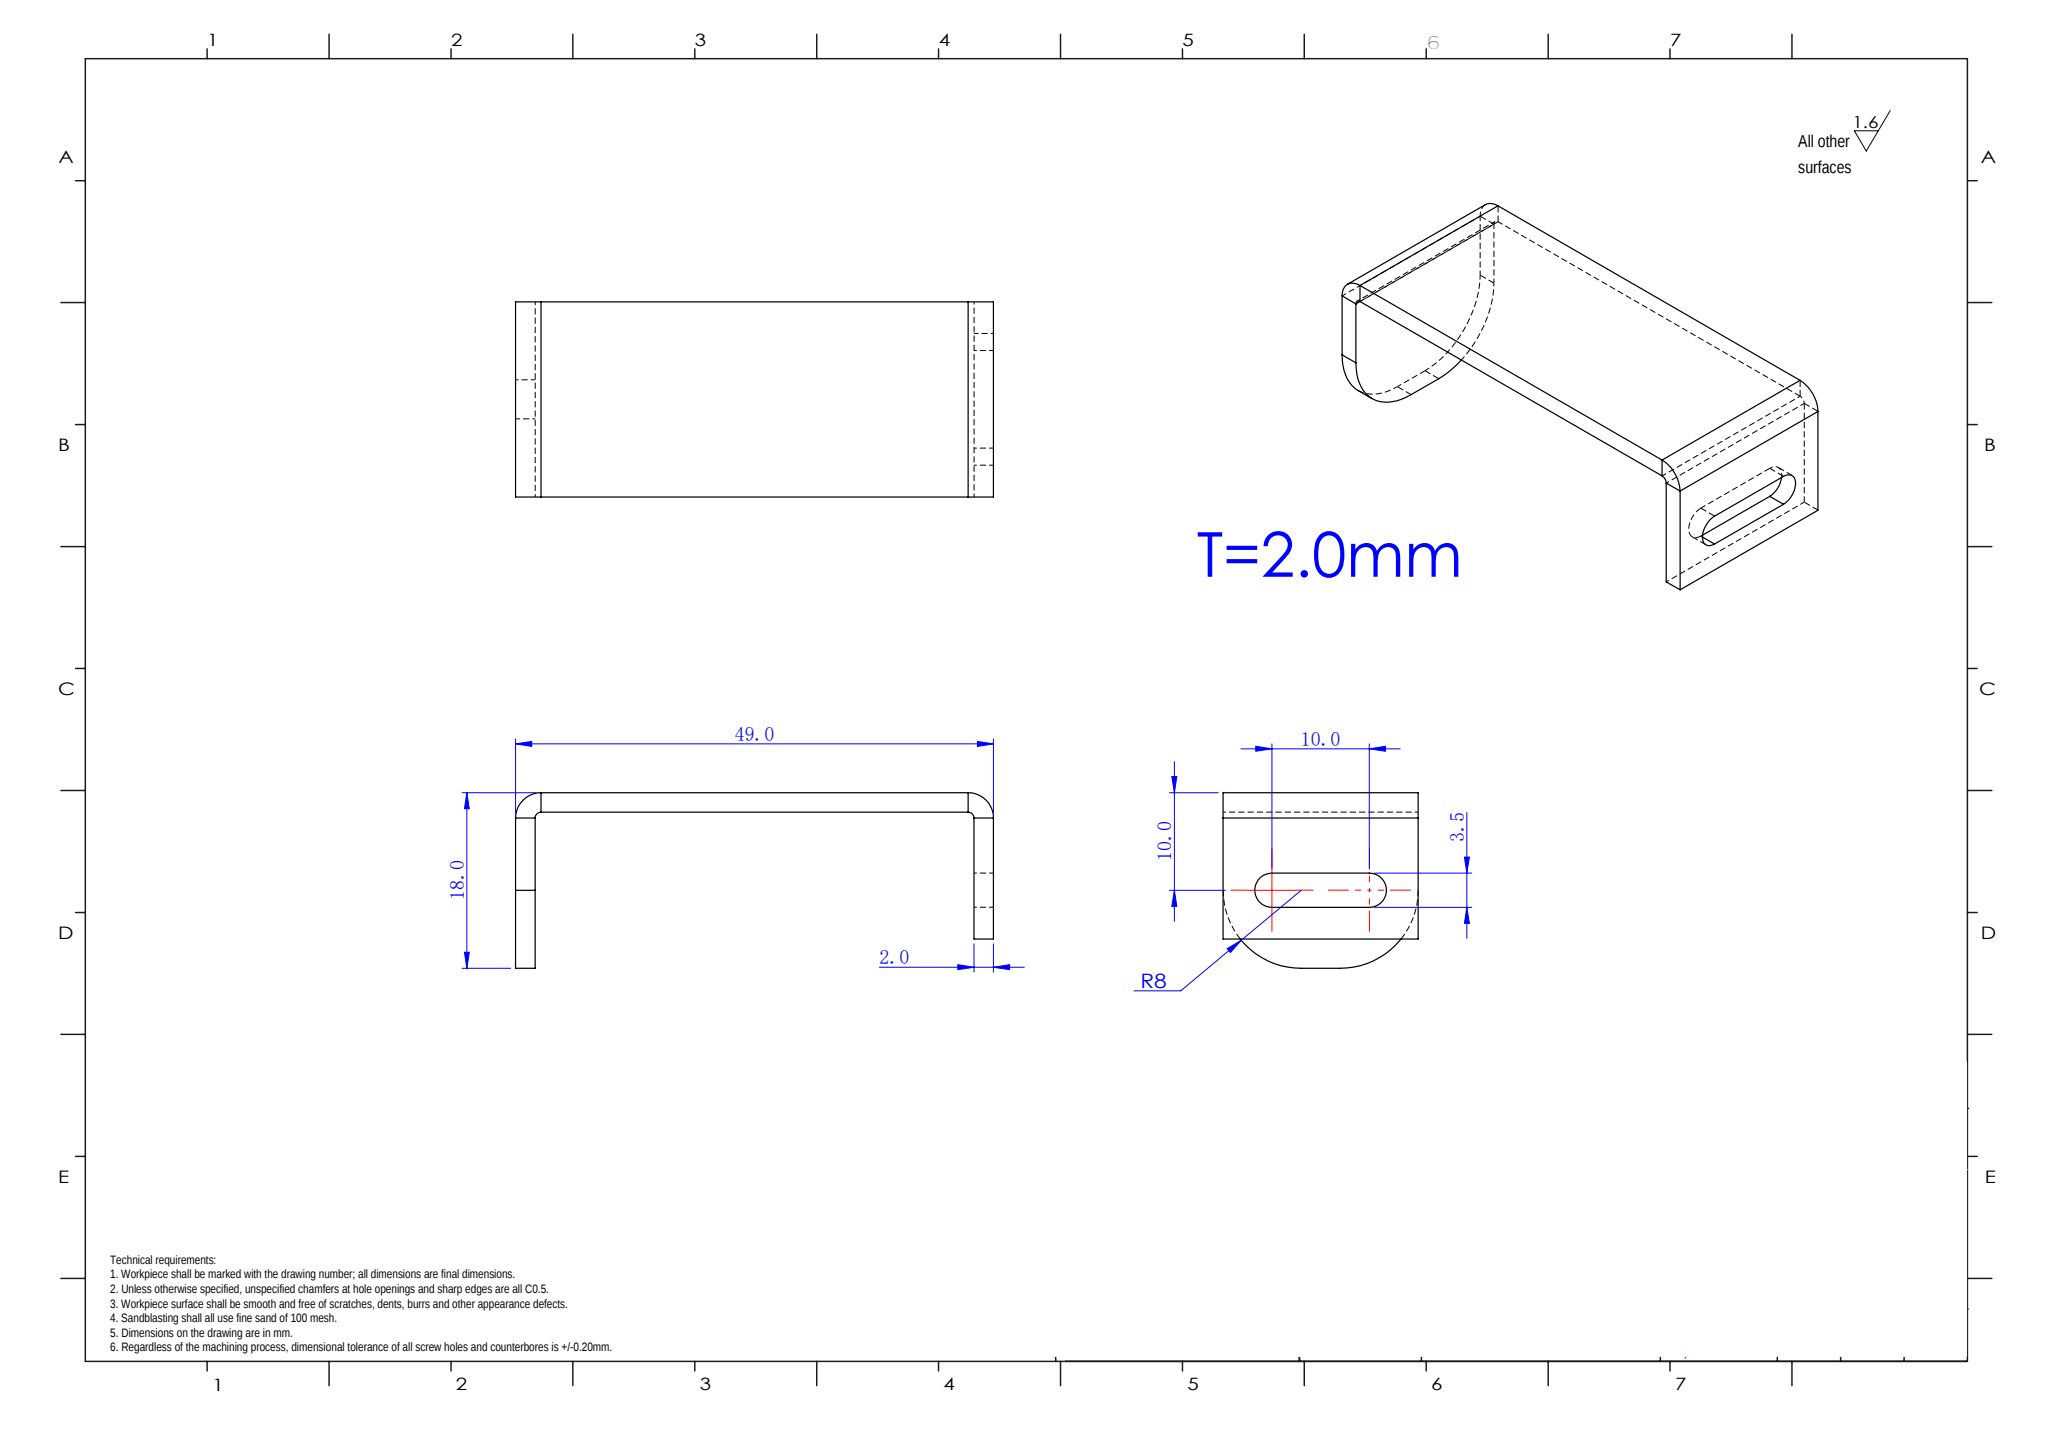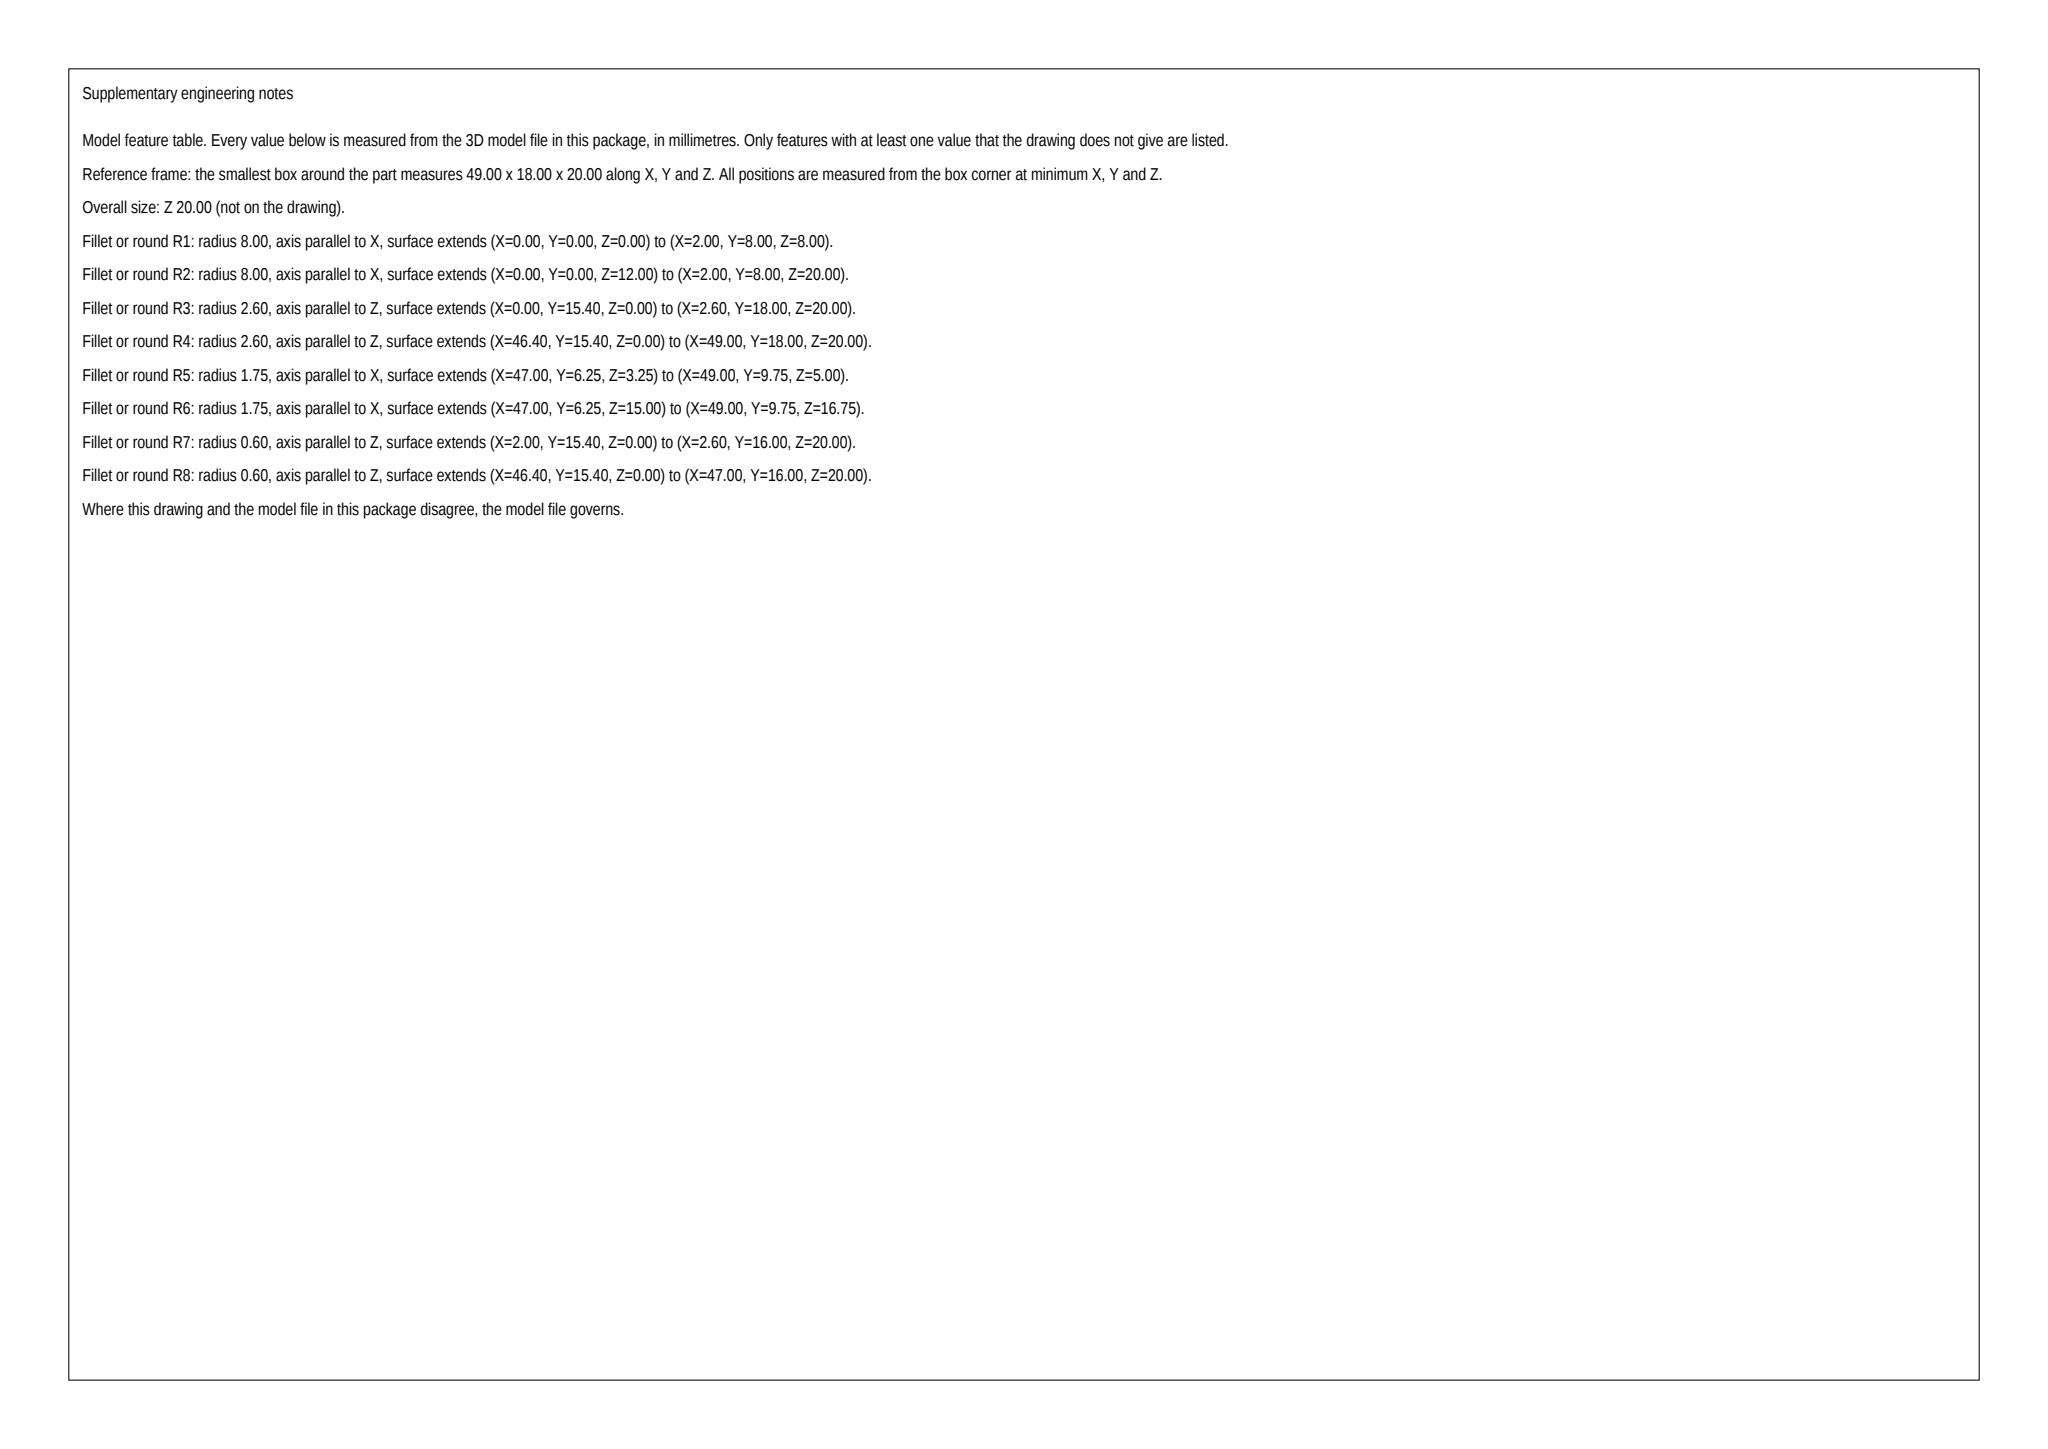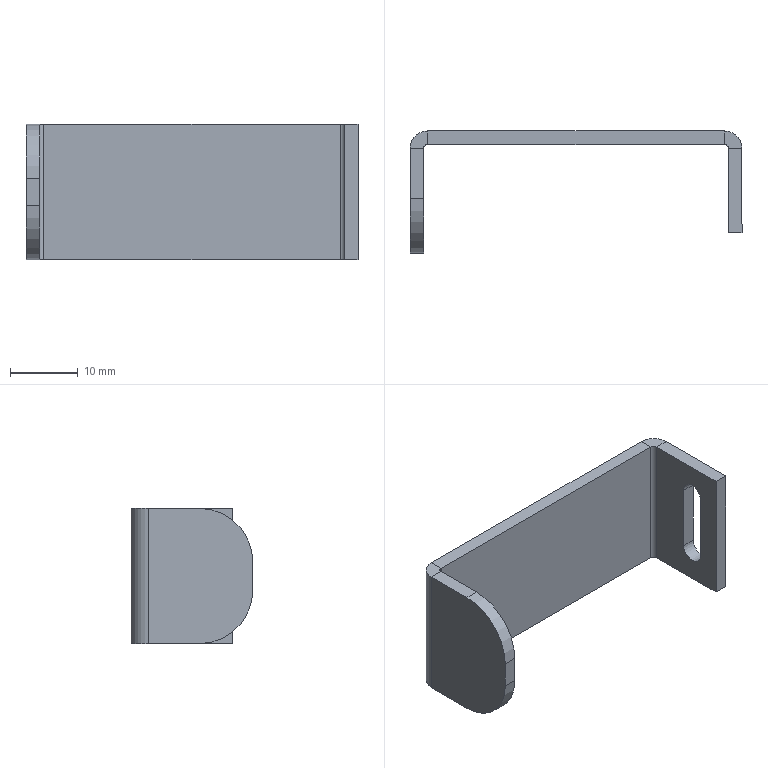Part | SolidWorks | mm | 1 solid | 28 faces | box 49 x 18 x 20 mm | volume 2921 mm3 | plane 20 | cylinder 8 | commonest cylinder face diameters 5.2 x2 1.2 x2 16 x2 3.5 x2
STEP:
#1=CARTESIAN_POINT('',(-2.6,2.,20.));
#2=VERTEX_POINT('',#1);
#3=CARTESIAN_POINT('',(-2.6,2.,0.));
#4=VERTEX_POINT('',#3);
#5=CARTESIAN_POINT('',(-2.6,2.,20.));
#6=DIRECTION('',(0.,0.,-1.));
#7=VECTOR('',#6,1000.);
#8=LINE('',#5,#7);
#9=EDGE_CURVE('',#2,#4,#8,.T.);
#10=ORIENTED_EDGE('',*,*,#9,.T.);
#11=CARTESIAN_POINT('',(-46.4,2.,0.));
#12=VERTEX_POINT('',#11);
#13=CARTESIAN_POINT('',(-0.,2.,0.));
#14=DIRECTION('',(-1.,-0.,0.));
#15=VECTOR('',#14,1000.);
#16=LINE('',#13,#15);
#17=EDGE_CURVE('',#4,#12,#16,.T.);
#18=ORIENTED_EDGE('',*,*,#17,.T.);
#19=CARTESIAN_POINT('',(-46.4,2.,20.));
#20=VERTEX_POINT('',#19);
#21=CARTESIAN_POINT('',(-46.4,2.,0.));
#22=DIRECTION('',(0.,0.,1.));
#23=VECTOR('',#22,1000.);
#24=LINE('',#21,#23);
#25=EDGE_CURVE('',#12,#20,#24,.T.);
#26=ORIENTED_EDGE('',*,*,#25,.T.);
#27=CARTESIAN_POINT('',(-0.,2.,20.));
#28=DIRECTION('',(-1.,-0.,0.));
#29=VECTOR('',#28,1000.);
#30=LINE('',#27,#29);
#31=EDGE_CURVE('',#2,#20,#30,.T.);
#32=ORIENTED_EDGE('',*,*,#31,.F.);
#33=EDGE_LOOP('',(#10,#18,#26,#32));
#34=FACE_OUTER_BOUND('',#33,.T.);
#35=CARTESIAN_POINT('',(-0.,2.,20.));
#36=DIRECTION('',(0.,-1.,0.));
#37=DIRECTION('',(1.,0.,0.));
#38=AXIS2_PLACEMENT_3D('',#35,#36,#37);
#39=PLANE('',#38);
#40=ADVANCED_FACE('',(#34),#39,.F.);
#41=CARTESIAN_POINT('',(-2.6,-0.,0.));
#42=VERTEX_POINT('',#41);
#43=CARTESIAN_POINT('',(-46.4,-0.,0.));
#44=VERTEX_POINT('',#43);
#45=CARTESIAN_POINT('',(0.,0.,0.));
#46=DIRECTION('',(-1.,-0.,0.));
#47=VECTOR('',#46,1000.);
#48=LINE('',#45,#47);
#49=EDGE_CURVE('',#42,#44,#48,.T.);
#50=ORIENTED_EDGE('',*,*,#49,.F.);
#51=CARTESIAN_POINT('',(-2.6,-0.,20.));
#52=VERTEX_POINT('',#51);
#53=CARTESIAN_POINT('',(-2.6,0.,20.));
#54=DIRECTION('',(0.,0.,-1.));
#55=VECTOR('',#54,1000.);
#56=LINE('',#53,#55);
#57=EDGE_CURVE('',#52,#42,#56,.T.);
#58=ORIENTED_EDGE('',*,*,#57,.F.);
#59=CARTESIAN_POINT('',(-46.4,-0.,20.));
#60=VERTEX_POINT('',#59);
#61=CARTESIAN_POINT('',(0.,0.,20.));
#62=DIRECTION('',(-1.,-0.,0.));
#63=VECTOR('',#62,1000.);
#64=LINE('',#61,#63);
#65=EDGE_CURVE('',#52,#60,#64,.T.);
#66=ORIENTED_EDGE('',*,*,#65,.T.);
#67=CARTESIAN_POINT('',(-46.4,-0.,0.));
#68=DIRECTION('',(0.,0.,1.));
#69=VECTOR('',#68,1000.);
#70=LINE('',#67,#69);
#71=EDGE_CURVE('',#44,#60,#70,.T.);
#72=ORIENTED_EDGE('',*,*,#71,.F.);
#73=EDGE_LOOP('',(#50,#58,#66,#72));
#74=FACE_OUTER_BOUND('',#73,.T.);
#75=CARTESIAN_POINT('',(0.,0.,20.));
#76=DIRECTION('',(0.,-1.,0.));
#77=DIRECTION('',(1.,0.,0.));
#78=AXIS2_PLACEMENT_3D('',#75,#76,#77);
#79=PLANE('',#78);
#80=ADVANCED_FACE('',(#74),#79,.T.);
#81=CARTESIAN_POINT('',(-2.6,0.,20.));
#82=DIRECTION('',(0.,1.,0.));
#83=VECTOR('',#82,1000.);
#84=LINE('',#81,#83);
#85=EDGE_CURVE('',#52,#2,#84,.T.);
#86=ORIENTED_EDGE('',*,*,#85,.T.);
#87=ORIENTED_EDGE('',*,*,#31,.T.);
#88=CARTESIAN_POINT('',(-46.4,-0.,20.));
#89=DIRECTION('',(0.,1.,0.));
#90=VECTOR('',#89,1000.);
#91=LINE('',#88,#90);
#92=EDGE_CURVE('',#60,#20,#91,.T.);
#93=ORIENTED_EDGE('',*,*,#92,.F.);
#94=ORIENTED_EDGE('',*,*,#65,.F.);
#95=EDGE_LOOP('',(#86,#87,#93,#94));
#96=FACE_OUTER_BOUND('',#95,.T.);
#97=CARTESIAN_POINT('',(0.,0.,20.));
#98=DIRECTION('',(0.,0.,-1.));
#99=DIRECTION('',(-1.,0.,0.));
#100=AXIS2_PLACEMENT_3D('',#97,#98,#99);
#101=PLANE('',#100);
#102=ADVANCED_FACE('',(#96),#101,.F.);
#103=CARTESIAN_POINT('',(-2.6,0.,0.));
#104=DIRECTION('',(0.,1.,0.));
#105=VECTOR('',#104,1000.);
#106=LINE('',#103,#105);
#107=EDGE_CURVE('',#42,#4,#106,.T.);
#108=ORIENTED_EDGE('',*,*,#107,.F.);
#109=ORIENTED_EDGE('',*,*,#49,.T.);
#110=CARTESIAN_POINT('',(-46.4,-0.,0.));
#111=DIRECTION('',(0.,1.,0.));
#112=VECTOR('',#111,1000.);
#113=LINE('',#110,#112);
#114=EDGE_CURVE('',#44,#12,#113,.T.);
#115=ORIENTED_EDGE('',*,*,#114,.T.);
#116=ORIENTED_EDGE('',*,*,#17,.F.);
#117=EDGE_LOOP('',(#108,#109,#115,#116));
#118=FACE_OUTER_BOUND('',#117,.T.);
#119=CARTESIAN_POINT('',(0.,0.,0.));
#120=DIRECTION('',(0.,0.,-1.));
#121=DIRECTION('',(-1.,0.,0.));
#122=AXIS2_PLACEMENT_3D('',#119,#120,#121);
#123=PLANE('',#122);
#124=ADVANCED_FACE('',(#118),#123,.T.);
#125=CARTESIAN_POINT('',(-47.,-0.6,20.));
#126=VERTEX_POINT('',#125);
#127=CARTESIAN_POINT('',(-49.,-0.6,20.));
#128=VERTEX_POINT('',#127);
#129=CARTESIAN_POINT('',(-49.,-0.6,20.));
#130=DIRECTION('',(-1.,0.,0.));
#131=VECTOR('',#130,1000.);
#132=LINE('',#129,#131);
#133=EDGE_CURVE('',#126,#128,#132,.T.);
#134=ORIENTED_EDGE('',*,*,#133,.F.);
#135=CARTESIAN_POINT('',(-46.4,-0.6,20.));
#136=DIRECTION('',(0.,0.,1.));
#137=DIRECTION('',(-1.,-0.,0.));
#138=AXIS2_PLACEMENT_3D('',#135,#136,#137);
#139=CIRCLE('',#138,0.6);
#140=EDGE_CURVE('',#60,#126,#139,.T.);
#141=ORIENTED_EDGE('',*,*,#140,.F.);
#142=ORIENTED_EDGE('',*,*,#92,.T.);
#143=CARTESIAN_POINT('',(-46.4,-0.6,20.));
#144=DIRECTION('',(0.,0.,1.));
#145=DIRECTION('',(-1.,-0.,0.));
#146=AXIS2_PLACEMENT_3D('',#143,#144,#145);
#147=CIRCLE('',#146,2.6);
#148=EDGE_CURVE('',#20,#128,#147,.T.);
#149=ORIENTED_EDGE('',*,*,#148,.T.);
#150=EDGE_LOOP('',(#134,#141,#142,#149));
#151=FACE_OUTER_BOUND('',#150,.T.);
#152=CARTESIAN_POINT('',(-46.4,-0.6,20.));
#153=DIRECTION('',(0.,0.,1.));
#154=DIRECTION('',(1.,0.,0.));
#155=AXIS2_PLACEMENT_3D('',#152,#153,#154);
#156=PLANE('',#155);
#157=ADVANCED_FACE('',(#151),#156,.T.);
#158=CARTESIAN_POINT('',(-47.,-0.6,0.));
#159=VERTEX_POINT('',#158);
#160=CARTESIAN_POINT('',(-46.4,-0.6,0.));
#161=DIRECTION('',(0.,0.,-1.));
#162=DIRECTION('',(-1.,0.,0.));
#163=AXIS2_PLACEMENT_3D('',#160,#161,#162);
#164=CIRCLE('',#163,0.6);
#165=EDGE_CURVE('',#159,#44,#164,.T.);
#166=ORIENTED_EDGE('',*,*,#165,.F.);
#167=CARTESIAN_POINT('',(-49.,-0.6,0.));
#168=VERTEX_POINT('',#167);
#169=CARTESIAN_POINT('',(-47.,-0.6,0.));
#170=DIRECTION('',(-1.,0.,0.));
#171=VECTOR('',#170,1000.);
#172=LINE('',#169,#171);
#173=EDGE_CURVE('',#159,#168,#172,.T.);
#174=ORIENTED_EDGE('',*,*,#173,.T.);
#175=CARTESIAN_POINT('',(-46.4,-0.6,0.));
#176=DIRECTION('',(0.,0.,-1.));
#177=DIRECTION('',(-1.,0.,0.));
#178=AXIS2_PLACEMENT_3D('',#175,#176,#177);
#179=CIRCLE('',#178,2.6);
#180=EDGE_CURVE('',#168,#12,#179,.T.);
#181=ORIENTED_EDGE('',*,*,#180,.T.);
#182=ORIENTED_EDGE('',*,*,#114,.F.);
#183=EDGE_LOOP('',(#166,#174,#181,#182));
#184=FACE_OUTER_BOUND('',#183,.T.);
#185=CARTESIAN_POINT('',(-46.4,-0.6,0.));
#186=DIRECTION('',(0.,0.,1.));
#187=DIRECTION('',(1.,0.,0.));
#188=AXIS2_PLACEMENT_3D('',#185,#186,#187);
#189=PLANE('',#188);
#190=ADVANCED_FACE('',(#184),#189,.F.);
#191=ORIENTED_EDGE('',*,*,#25,.F.);
#192=ORIENTED_EDGE('',*,*,#180,.F.);
#193=CARTESIAN_POINT('',(-49.,-0.6,0.));
#194=DIRECTION('',(0.,0.,-1.));
#195=VECTOR('',#194,1000.);
#196=LINE('',#193,#195);
#197=EDGE_CURVE('',#128,#168,#196,.T.);
#198=ORIENTED_EDGE('',*,*,#197,.F.);
#199=ORIENTED_EDGE('',*,*,#148,.F.);
#200=EDGE_LOOP('',(#191,#192,#198,#199));
#201=FACE_OUTER_BOUND('',#200,.T.);
#202=CARTESIAN_POINT('',(-46.4,-0.6,0.));
#203=DIRECTION('',(0.,0.,-1.));
#204=DIRECTION('',(-1.,0.,0.));
#205=AXIS2_PLACEMENT_3D('',#202,#203,#204);
#206=CYLINDRICAL_SURFACE('',#205,2.6);
#207=ADVANCED_FACE('',(#201),#206,.T.);
#208=ORIENTED_EDGE('',*,*,#71,.T.);
#209=ORIENTED_EDGE('',*,*,#140,.T.);
#210=CARTESIAN_POINT('',(-47.,-0.6,20.));
#211=DIRECTION('',(0.,0.,-1.));
#212=VECTOR('',#211,1000.);
#213=LINE('',#210,#212);
#214=EDGE_CURVE('',#126,#159,#213,.T.);
#215=ORIENTED_EDGE('',*,*,#214,.T.);
#216=ORIENTED_EDGE('',*,*,#165,.T.);
#217=EDGE_LOOP('',(#208,#209,#215,#216));
#218=FACE_OUTER_BOUND('',#217,.T.);
#219=CARTESIAN_POINT('',(-46.4,-0.6,0.));
#220=DIRECTION('',(0.,0.,-1.));
#221=DIRECTION('',(-1.,0.,0.));
#222=AXIS2_PLACEMENT_3D('',#219,#220,#221);
#223=CYLINDRICAL_SURFACE('',#222,0.6);
#224=ADVANCED_FACE('',(#218),#223,.F.);
#225=CARTESIAN_POINT('',(-47.,-8.,0.));
#226=VERTEX_POINT('',#225);
#227=CARTESIAN_POINT('',(-47.,0.,0.));
#228=DIRECTION('',(0.,1.,0.));
#229=VECTOR('',#228,1000.);
#230=LINE('',#227,#229);
#231=EDGE_CURVE('',#226,#159,#230,.T.);
#232=ORIENTED_EDGE('',*,*,#231,.F.);
#233=CARTESIAN_POINT('',(-49.,-8.,0.));
#234=VERTEX_POINT('',#233);
#235=CARTESIAN_POINT('',(-49.,-8.,0.));
#236=DIRECTION('',(-1.,0.,0.));
#237=VECTOR('',#236,1000.);
#238=LINE('',#235,#237);
#239=EDGE_CURVE('',#226,#234,#238,.T.);
#240=ORIENTED_EDGE('',*,*,#239,.T.);
#241=CARTESIAN_POINT('',(-49.,0.,0.));
#242=DIRECTION('',(0.,1.,0.));
#243=VECTOR('',#242,1000.);
#244=LINE('',#241,#243);
#245=EDGE_CURVE('',#234,#168,#244,.T.);
#246=ORIENTED_EDGE('',*,*,#245,.T.);
#247=ORIENTED_EDGE('',*,*,#173,.F.);
#248=EDGE_LOOP('',(#232,#240,#246,#247));
#249=FACE_OUTER_BOUND('',#248,.T.);
#250=CARTESIAN_POINT('',(-49.,0.,0.));
#251=DIRECTION('',(0.,0.,-1.));
#252=DIRECTION('',(-1.,0.,0.));
#253=AXIS2_PLACEMENT_3D('',#250,#251,#252);
#254=PLANE('',#253);
#255=ADVANCED_FACE('',(#249),#254,.T.);
#256=CARTESIAN_POINT('',(-49.,-8.,20.));
#257=VERTEX_POINT('',#256);
#258=CARTESIAN_POINT('',(-49.,-16.,20.));
#259=DIRECTION('',(-0.,-1.,0.));
#260=VECTOR('',#259,1000.);
#261=LINE('',#258,#260);
#262=EDGE_CURVE('',#128,#257,#261,.T.);
#263=ORIENTED_EDGE('',*,*,#262,.T.);
#264=CARTESIAN_POINT('',(-47.,-8.,20.));
#265=VERTEX_POINT('',#264);
#266=CARTESIAN_POINT('',(-49.,-8.,20.));
#267=DIRECTION('',(1.,-0.,0.));
#268=VECTOR('',#267,1000.);
#269=LINE('',#266,#268);
#270=EDGE_CURVE('',#257,#265,#269,.T.);
#271=ORIENTED_EDGE('',*,*,#270,.T.);
#272=CARTESIAN_POINT('',(-47.,0.,20.));
#273=DIRECTION('',(-0.,-1.,0.));
#274=VECTOR('',#273,1000.);
#275=LINE('',#272,#274);
#276=EDGE_CURVE('',#126,#265,#275,.T.);
#277=ORIENTED_EDGE('',*,*,#276,.F.);
#278=ORIENTED_EDGE('',*,*,#133,.T.);
#279=EDGE_LOOP('',(#263,#271,#277,#278));
#280=FACE_OUTER_BOUND('',#279,.T.);
#281=CARTESIAN_POINT('',(-49.,-16.,20.));
#282=DIRECTION('',(0.,0.,1.));
#283=DIRECTION('',(1.,0.,0.));
#284=AXIS2_PLACEMENT_3D('',#281,#282,#283);
#285=PLANE('',#284);
#286=ADVANCED_FACE('',(#280),#285,.T.);
#287=CARTESIAN_POINT('',(-49.,-16.,12.));
#288=VERTEX_POINT('',#287);
#289=CARTESIAN_POINT('',(-49.,-16.,8.));
#290=VERTEX_POINT('',#289);
#291=CARTESIAN_POINT('',(-49.,-16.,0.));
#292=DIRECTION('',(0.,0.,-1.));
#293=VECTOR('',#292,1000.);
#294=LINE('',#291,#293);
#295=EDGE_CURVE('',#288,#290,#294,.T.);
#296=ORIENTED_EDGE('',*,*,#295,.F.);
#297=CARTESIAN_POINT('',(-49.,-8.,12.));
#298=DIRECTION('',(-1.,0.,0.));
#299=DIRECTION('',(-0.,-1.,0.));
#300=AXIS2_PLACEMENT_3D('',#297,#298,#299);
#301=CIRCLE('',#300,8.);
#302=EDGE_CURVE('',#288,#257,#301,.T.);
#303=ORIENTED_EDGE('',*,*,#302,.T.);
#304=ORIENTED_EDGE('',*,*,#262,.F.);
#305=ORIENTED_EDGE('',*,*,#197,.T.);
#306=ORIENTED_EDGE('',*,*,#245,.F.);
#307=CARTESIAN_POINT('',(-49.,-8.,8.));
#308=DIRECTION('',(-1.,0.,0.));
#309=DIRECTION('',(-0.,-1.,0.));
#310=AXIS2_PLACEMENT_3D('',#307,#308,#309);
#311=CIRCLE('',#310,8.);
#312=EDGE_CURVE('',#234,#290,#311,.T.);
#313=ORIENTED_EDGE('',*,*,#312,.T.);
#314=EDGE_LOOP('',(#296,#303,#304,#305,#306,#313));
#315=FACE_OUTER_BOUND('',#314,.T.);
#316=CARTESIAN_POINT('',(-49.,0.,0.));
#317=DIRECTION('',(-1.,0.,0.));
#318=DIRECTION('',(-0.,-1.,0.));
#319=AXIS2_PLACEMENT_3D('',#316,#317,#318);
#320=PLANE('',#319);
#321=ADVANCED_FACE('',(#315),#320,.T.);
#322=ORIENTED_EDGE('',*,*,#276,.T.);
#323=CARTESIAN_POINT('',(-47.,-16.,12.));
#324=VERTEX_POINT('',#323);
#325=CARTESIAN_POINT('',(-47.,-8.,12.));
#326=DIRECTION('',(1.,-0.,0.));
#327=DIRECTION('',(-0.,-1.,0.));
#328=AXIS2_PLACEMENT_3D('',#325,#326,#327);
#329=CIRCLE('',#328,8.);
#330=EDGE_CURVE('',#265,#324,#329,.T.);
#331=ORIENTED_EDGE('',*,*,#330,.T.);
#332=CARTESIAN_POINT('',(-47.,-16.,8.));
#333=VERTEX_POINT('',#332);
#334=CARTESIAN_POINT('',(-47.,-16.,0.));
#335=DIRECTION('',(0.,0.,-1.));
#336=VECTOR('',#335,1000.);
#337=LINE('',#334,#336);
#338=EDGE_CURVE('',#324,#333,#337,.T.);
#339=ORIENTED_EDGE('',*,*,#338,.T.);
#340=CARTESIAN_POINT('',(-47.,-8.,8.));
#341=DIRECTION('',(1.,-0.,0.));
#342=DIRECTION('',(-0.,-1.,0.));
#343=AXIS2_PLACEMENT_3D('',#340,#341,#342);
#344=CIRCLE('',#343,8.);
#345=EDGE_CURVE('',#333,#226,#344,.T.);
#346=ORIENTED_EDGE('',*,*,#345,.T.);
#347=ORIENTED_EDGE('',*,*,#231,.T.);
#348=ORIENTED_EDGE('',*,*,#214,.F.);
#349=EDGE_LOOP('',(#322,#331,#339,#346,#347,#348));
#350=FACE_OUTER_BOUND('',#349,.T.);
#351=CARTESIAN_POINT('',(-47.,0.,0.));
#352=DIRECTION('',(-1.,0.,0.));
#353=DIRECTION('',(-0.,-1.,0.));
#354=AXIS2_PLACEMENT_3D('',#351,#352,#353);
#355=PLANE('',#354);
#356=ADVANCED_FACE('',(#350),#355,.F.);
#357=ORIENTED_EDGE('',*,*,#338,.F.);
#358=CARTESIAN_POINT('',(-49.,-16.,12.));
#359=DIRECTION('',(-1.,0.,0.));
#360=VECTOR('',#359,1000.);
#361=LINE('',#358,#360);
#362=EDGE_CURVE('',#324,#288,#361,.T.);
#363=ORIENTED_EDGE('',*,*,#362,.T.);
#364=ORIENTED_EDGE('',*,*,#295,.T.);
#365=CARTESIAN_POINT('',(-49.,-16.,8.));
#366=DIRECTION('',(1.,-0.,0.));
#367=VECTOR('',#366,1000.);
#368=LINE('',#365,#367);
#369=EDGE_CURVE('',#290,#333,#368,.T.);
#370=ORIENTED_EDGE('',*,*,#369,.T.);
#371=EDGE_LOOP('',(#357,#363,#364,#370));
#372=FACE_OUTER_BOUND('',#371,.T.);
#373=CARTESIAN_POINT('',(-49.,-16.,0.));
#374=DIRECTION('',(-0.,-1.,0.));
#375=DIRECTION('',(1.,-0.,0.));
#376=AXIS2_PLACEMENT_3D('',#373,#374,#375);
#377=PLANE('',#376);
#378=ADVANCED_FACE('',(#372),#377,.T.);
#379=ORIENTED_EDGE('',*,*,#302,.F.);
#380=ORIENTED_EDGE('',*,*,#362,.F.);
#381=ORIENTED_EDGE('',*,*,#330,.F.);
#382=ORIENTED_EDGE('',*,*,#270,.F.);
#383=EDGE_LOOP('',(#379,#380,#381,#382));
#384=FACE_OUTER_BOUND('',#383,.T.);
#385=CARTESIAN_POINT('',(-49.,-8.,12.));
#386=DIRECTION('',(1.,-0.,0.));
#387=DIRECTION('',(0.,1.,0.));
#388=AXIS2_PLACEMENT_3D('',#385,#386,#387);
#389=CYLINDRICAL_SURFACE('',#388,8.);
#390=ADVANCED_FACE('',(#384),#389,.T.);
#391=ORIENTED_EDGE('',*,*,#312,.F.);
#392=ORIENTED_EDGE('',*,*,#239,.F.);
#393=ORIENTED_EDGE('',*,*,#345,.F.);
#394=ORIENTED_EDGE('',*,*,#369,.F.);
#395=EDGE_LOOP('',(#391,#392,#393,#394));
#396=FACE_OUTER_BOUND('',#395,.T.);
#397=CARTESIAN_POINT('',(-49.,-8.,8.));
#398=DIRECTION('',(1.,-0.,0.));
#399=DIRECTION('',(0.,1.,0.));
#400=AXIS2_PLACEMENT_3D('',#397,#398,#399);
#401=CYLINDRICAL_SURFACE('',#400,8.);
#402=ADVANCED_FACE('',(#396),#401,.T.);
#403=CARTESIAN_POINT('',(-2.,-0.6,0.));
#404=VERTEX_POINT('',#403);
#405=CARTESIAN_POINT('',(0.,-0.6,0.));
#406=VERTEX_POINT('',#405);
#407=CARTESIAN_POINT('',(0.,-0.6,0.));
#408=DIRECTION('',(1.,0.,0.));
#409=VECTOR('',#408,1000.);
#410=LINE('',#407,#409);
#411=EDGE_CURVE('',#404,#406,#410,.T.);
#412=ORIENTED_EDGE('',*,*,#411,.F.);
#413=CARTESIAN_POINT('',(-2.6,-0.6,0.));
#414=DIRECTION('',(0.,0.,-1.));
#415=DIRECTION('',(1.,-0.,0.));
#416=AXIS2_PLACEMENT_3D('',#413,#414,#415);
#417=CIRCLE('',#416,0.6);
#418=EDGE_CURVE('',#42,#404,#417,.T.);
#419=ORIENTED_EDGE('',*,*,#418,.F.);
#420=ORIENTED_EDGE('',*,*,#107,.T.);
#421=CARTESIAN_POINT('',(-2.6,-0.6,0.));
#422=DIRECTION('',(0.,0.,-1.));
#423=DIRECTION('',(1.,-0.,0.));
#424=AXIS2_PLACEMENT_3D('',#421,#422,#423);
#425=CIRCLE('',#424,2.6);
#426=EDGE_CURVE('',#4,#406,#425,.T.);
#427=ORIENTED_EDGE('',*,*,#426,.T.);
#428=EDGE_LOOP('',(#412,#419,#420,#427));
#429=FACE_OUTER_BOUND('',#428,.T.);
#430=CARTESIAN_POINT('',(-2.6,-0.6,0.));
#431=DIRECTION('',(0.,0.,-1.));
#432=DIRECTION('',(-1.,0.,0.));
#433=AXIS2_PLACEMENT_3D('',#430,#431,#432);
#434=PLANE('',#433);
#435=ADVANCED_FACE('',(#429),#434,.T.);
#436=CARTESIAN_POINT('',(-2.,-0.6,20.));
#437=VERTEX_POINT('',#436);
#438=CARTESIAN_POINT('',(-2.6,-0.6,20.));
#439=DIRECTION('',(0.,0.,1.));
#440=DIRECTION('',(1.,0.,0.));
#441=AXIS2_PLACEMENT_3D('',#438,#439,#440);
#442=CIRCLE('',#441,0.6);
#443=EDGE_CURVE('',#437,#52,#442,.T.);
#444=ORIENTED_EDGE('',*,*,#443,.F.);
#445=CARTESIAN_POINT('',(0.,-0.6,20.));
#446=VERTEX_POINT('',#445);
#447=CARTESIAN_POINT('',(-2.,-0.6,20.));
#448=DIRECTION('',(1.,0.,0.));
#449=VECTOR('',#448,1000.);
#450=LINE('',#447,#449);
#451=EDGE_CURVE('',#437,#446,#450,.T.);
#452=ORIENTED_EDGE('',*,*,#451,.T.);
#453=CARTESIAN_POINT('',(-2.6,-0.6,20.));
#454=DIRECTION('',(0.,0.,1.));
#455=DIRECTION('',(1.,0.,0.));
#456=AXIS2_PLACEMENT_3D('',#453,#454,#455);
#457=CIRCLE('',#456,2.6);
#458=EDGE_CURVE('',#446,#2,#457,.T.);
#459=ORIENTED_EDGE('',*,*,#458,.T.);
#460=ORIENTED_EDGE('',*,*,#85,.F.);
#461=EDGE_LOOP('',(#444,#452,#459,#460));
#462=FACE_OUTER_BOUND('',#461,.T.);
#463=CARTESIAN_POINT('',(-2.6,-0.6,20.));
#464=DIRECTION('',(0.,0.,-1.));
#465=DIRECTION('',(-1.,0.,0.));
#466=AXIS2_PLACEMENT_3D('',#463,#464,#465);
#467=PLANE('',#466);
#468=ADVANCED_FACE('',(#462),#467,.F.);
#469=ORIENTED_EDGE('',*,*,#9,.F.);
#470=ORIENTED_EDGE('',*,*,#458,.F.);
#471=CARTESIAN_POINT('',(0.,-0.6,-0.));
#472=DIRECTION('',(0.,-0.,1.));
#473=VECTOR('',#472,1000.);
#474=LINE('',#471,#473);
#475=EDGE_CURVE('',#406,#446,#474,.T.);
#476=ORIENTED_EDGE('',*,*,#475,.F.);
#477=ORIENTED_EDGE('',*,*,#426,.F.);
#478=EDGE_LOOP('',(#469,#470,#476,#477));
#479=FACE_OUTER_BOUND('',#478,.T.);
#480=CARTESIAN_POINT('',(-2.6,-0.6,20.));
#481=DIRECTION('',(0.,0.,1.));
#482=DIRECTION('',(1.,0.,0.));
#483=AXIS2_PLACEMENT_3D('',#480,#481,#482);
#484=CYLINDRICAL_SURFACE('',#483,2.6);
#485=ADVANCED_FACE('',(#479),#484,.T.);
#486=ORIENTED_EDGE('',*,*,#57,.T.);
#487=ORIENTED_EDGE('',*,*,#418,.T.);
#488=CARTESIAN_POINT('',(-2.,-0.6,0.));
#489=DIRECTION('',(0.,-0.,1.));
#490=VECTOR('',#489,1000.);
#491=LINE('',#488,#490);
#492=EDGE_CURVE('',#404,#437,#491,.T.);
#493=ORIENTED_EDGE('',*,*,#492,.T.);
#494=ORIENTED_EDGE('',*,*,#443,.T.);
#495=EDGE_LOOP('',(#486,#487,#493,#494));
#496=FACE_OUTER_BOUND('',#495,.T.);
#497=CARTESIAN_POINT('',(-2.6,-0.6,20.));
#498=DIRECTION('',(0.,0.,1.));
#499=DIRECTION('',(1.,0.,0.));
#500=AXIS2_PLACEMENT_3D('',#497,#498,#499);
#501=CYLINDRICAL_SURFACE('',#500,0.6);
#502=ADVANCED_FACE('',(#496),#501,.F.);
#503=CARTESIAN_POINT('',(0.,-13.,20.));
#504=VERTEX_POINT('',#503);
#505=CARTESIAN_POINT('',(0.,0.,20.));
#506=DIRECTION('',(-0.,1.,0.));
#507=VECTOR('',#506,1000.);
#508=LINE('',#505,#507);
#509=EDGE_CURVE('',#504,#446,#508,.T.);
#510=ORIENTED_EDGE('',*,*,#509,.T.);
#511=ORIENTED_EDGE('',*,*,#451,.F.);
#512=CARTESIAN_POINT('',(-2.,-13.,20.));
#513=VERTEX_POINT('',#512);
#514=CARTESIAN_POINT('',(-2.,-0.,20.));
#515=DIRECTION('',(-0.,1.,0.));
#516=VECTOR('',#515,1000.);
#517=LINE('',#514,#516);
#518=EDGE_CURVE('',#513,#437,#517,.T.);
#519=ORIENTED_EDGE('',*,*,#518,.F.);
#520=CARTESIAN_POINT('',(0.,-13.,20.));
#521=DIRECTION('',(-1.,-0.,0.));
#522=VECTOR('',#521,1000.);
#523=LINE('',#520,#522);
#524=EDGE_CURVE('',#504,#513,#523,.T.);
#525=ORIENTED_EDGE('',*,*,#524,.F.);
#526=EDGE_LOOP('',(#510,#511,#519,#525));
#527=FACE_OUTER_BOUND('',#526,.T.);
#528=CARTESIAN_POINT('',(0.,0.,20.));
#529=DIRECTION('',(0.,0.,1.));
#530=DIRECTION('',(1.,0.,0.));
#531=AXIS2_PLACEMENT_3D('',#528,#529,#530);
#532=PLANE('',#531);
#533=ADVANCED_FACE('',(#527),#532,.T.);
#534=CARTESIAN_POINT('',(-2.,-13.,0.));
#535=VERTEX_POINT('',#534);
#536=CARTESIAN_POINT('',(-2.,-0.,0.));
#537=DIRECTION('',(0.,-1.,0.));
#538=VECTOR('',#537,1000.);
#539=LINE('',#536,#538);
#540=EDGE_CURVE('',#404,#535,#539,.T.);
#541=ORIENTED_EDGE('',*,*,#540,.F.);
#542=ORIENTED_EDGE('',*,*,#411,.T.);
#543=CARTESIAN_POINT('',(0.,-13.,0.));
#544=VERTEX_POINT('',#543);
#545=CARTESIAN_POINT('',(0.,-13.,0.));
#546=DIRECTION('',(0.,-1.,0.));
#547=VECTOR('',#546,1000.);
#548=LINE('',#545,#547);
#549=EDGE_CURVE('',#406,#544,#548,.T.);
#550=ORIENTED_EDGE('',*,*,#549,.T.);
#551=CARTESIAN_POINT('',(0.,-13.,0.));
#552=DIRECTION('',(-1.,-0.,0.));
#553=VECTOR('',#552,1000.);
#554=LINE('',#551,#553);
#555=EDGE_CURVE('',#544,#535,#554,.T.);
#556=ORIENTED_EDGE('',*,*,#555,.T.);
#557=EDGE_LOOP('',(#541,#542,#550,#556));
#558=FACE_OUTER_BOUND('',#557,.T.);
#559=CARTESIAN_POINT('',(0.,-13.,0.));
#560=DIRECTION('',(0.,0.,-1.));
#561=DIRECTION('',(-1.,0.,0.));
#562=AXIS2_PLACEMENT_3D('',#559,#560,#561);
#563=PLANE('',#562);
#564=ADVANCED_FACE('',(#558),#563,.T.);
#565=CARTESIAN_POINT('',(0.,-6.25,15.));
#566=VERTEX_POINT('',#565);
#567=CARTESIAN_POINT('',(0.,-9.75,15.));
#568=VERTEX_POINT('',#567);
#569=CARTESIAN_POINT('',(0.,-8.,15.));
#570=DIRECTION('',(1.,0.,0.));
#571=DIRECTION('',(-0.,1.,0.));
#572=AXIS2_PLACEMENT_3D('',#569,#570,#571);
#573=CIRCLE('',#572,1.75);
#574=EDGE_CURVE('',#566,#568,#573,.T.);
#575=ORIENTED_EDGE('',*,*,#574,.F.);
#576=CARTESIAN_POINT('',(0.,-6.25,5.));
#577=VERTEX_POINT('',#576);
#578=CARTESIAN_POINT('',(0.,-6.25,15.));
#579=DIRECTION('',(-0.,0.,1.));
#580=VECTOR('',#579,1000.);
#581=LINE('',#578,#580);
#582=EDGE_CURVE('',#577,#566,#581,.T.);
#583=ORIENTED_EDGE('',*,*,#582,.F.);
#584=CARTESIAN_POINT('',(0.,-9.75,5.));
#585=VERTEX_POINT('',#584);
#586=CARTESIAN_POINT('',(0.,-8.,5.));
#587=DIRECTION('',(1.,0.,0.));
#588=DIRECTION('',(-0.,1.,0.));
#589=AXIS2_PLACEMENT_3D('',#586,#587,#588);
#590=CIRCLE('',#589,1.75);
#591=EDGE_CURVE('',#585,#577,#590,.T.);
#592=ORIENTED_EDGE('',*,*,#591,.F.);
#593=CARTESIAN_POINT('',(0.,-9.75,15.));
#594=DIRECTION('',(-0.,0.,-1.));
#595=VECTOR('',#594,1000.);
#596=LINE('',#593,#595);
#597=EDGE_CURVE('',#568,#585,#596,.T.);
#598=ORIENTED_EDGE('',*,*,#597,.F.);
#599=EDGE_LOOP('',(#575,#583,#592,#598));
#600=FACE_BOUND('',#599,.T.);
#601=ORIENTED_EDGE('',*,*,#549,.F.);
#602=ORIENTED_EDGE('',*,*,#475,.T.);
#603=ORIENTED_EDGE('',*,*,#509,.F.);
#604=CARTESIAN_POINT('',(0.,-13.,20.));
#605=DIRECTION('',(0.,0.,1.));
#606=VECTOR('',#605,1000.);
#607=LINE('',#604,#606);
#608=EDGE_CURVE('',#544,#504,#607,.T.);
#609=ORIENTED_EDGE('',*,*,#608,.F.);
#610=EDGE_LOOP('',(#601,#602,#603,#609));
#611=FACE_OUTER_BOUND('',#610,.T.);
#612=CARTESIAN_POINT('',(0.,0.,0.));
#613=DIRECTION('',(1.,0.,0.));
#614=DIRECTION('',(-0.,1.,0.));
#615=AXIS2_PLACEMENT_3D('',#612,#613,#614);
#616=PLANE('',#615);
#617=ADVANCED_FACE('',(#600,#611),#616,.T.);
#618=CARTESIAN_POINT('',(-2.,-6.25,5.));
#619=VERTEX_POINT('',#618);
#620=CARTESIAN_POINT('',(-2.,-6.25,15.));
#621=VERTEX_POINT('',#620);
#622=CARTESIAN_POINT('',(-2.,-6.25,0.));
#623=DIRECTION('',(-0.,0.,1.));
#624=VECTOR('',#623,1000.);
#625=LINE('',#622,#624);
#626=EDGE_CURVE('',#619,#621,#625,.T.);
#627=ORIENTED_EDGE('',*,*,#626,.T.);
#628=CARTESIAN_POINT('',(-2.,-9.75,15.));
#629=VERTEX_POINT('',#628);
#630=CARTESIAN_POINT('',(-2.,-8.,15.));
#631=DIRECTION('',(1.,0.,0.));
#632=DIRECTION('',(-0.,1.,0.));
#633=AXIS2_PLACEMENT_3D('',#630,#631,#632);
#634=CIRCLE('',#633,1.75);
#635=EDGE_CURVE('',#621,#629,#634,.T.);
#636=ORIENTED_EDGE('',*,*,#635,.T.);
#637=CARTESIAN_POINT('',(-2.,-9.75,5.));
#638=VERTEX_POINT('',#637);
#639=CARTESIAN_POINT('',(-2.,-9.75,-0.));
#640=DIRECTION('',(-0.,0.,-1.));
#641=VECTOR('',#640,1000.);
#642=LINE('',#639,#641);
#643=EDGE_CURVE('',#629,#638,#642,.T.);
#644=ORIENTED_EDGE('',*,*,#643,.T.);
#645=CARTESIAN_POINT('',(-2.,-8.,5.));
#646=DIRECTION('',(1.,0.,0.));
#647=DIRECTION('',(-0.,1.,0.));
#648=AXIS2_PLACEMENT_3D('',#645,#646,#647);
#649=CIRCLE('',#648,1.75);
#650=EDGE_CURVE('',#638,#619,#649,.T.);
#651=ORIENTED_EDGE('',*,*,#650,.T.);
#652=EDGE_LOOP('',(#627,#636,#644,#651));
#653=FACE_BOUND('',#652,.T.);
#654=ORIENTED_EDGE('',*,*,#492,.F.);
#655=ORIENTED_EDGE('',*,*,#540,.T.);
#656=CARTESIAN_POINT('',(-2.,-13.,0.));
#657=DIRECTION('',(0.,0.,1.));
#658=VECTOR('',#657,1000.);
#659=LINE('',#656,#658);
#660=EDGE_CURVE('',#535,#513,#659,.T.);
#661=ORIENTED_EDGE('',*,*,#660,.T.);
#662=ORIENTED_EDGE('',*,*,#518,.T.);
#663=EDGE_LOOP('',(#654,#655,#661,#662));
#664=FACE_OUTER_BOUND('',#663,.T.);
#665=CARTESIAN_POINT('',(-2.,-0.,0.));
#666=DIRECTION('',(1.,0.,0.));
#667=DIRECTION('',(-0.,1.,0.));
#668=AXIS2_PLACEMENT_3D('',#665,#666,#667);
#669=PLANE('',#668);
#670=ADVANCED_FACE('',(#653,#664),#669,.F.);
#671=ORIENTED_EDGE('',*,*,#660,.F.);
#672=ORIENTED_EDGE('',*,*,#555,.F.);
#673=ORIENTED_EDGE('',*,*,#608,.T.);
#674=ORIENTED_EDGE('',*,*,#524,.T.);
#675=EDGE_LOOP('',(#671,#672,#673,#674));
#676=FACE_OUTER_BOUND('',#675,.T.);
#677=CARTESIAN_POINT('',(0.,-13.,20.));
#678=DIRECTION('',(0.,-1.,0.));
#679=DIRECTION('',(1.,0.,0.));
#680=AXIS2_PLACEMENT_3D('',#677,#678,#679);
#681=PLANE('',#680);
#682=ADVANCED_FACE('',(#676),#681,.T.);
#683=CARTESIAN_POINT('',(-10.,-6.25,15.));
#684=DIRECTION('',(1.,0.,0.));
#685=VECTOR('',#684,1000.);
#686=LINE('',#683,#685);
#687=EDGE_CURVE('',#621,#566,#686,.T.);
#688=ORIENTED_EDGE('',*,*,#687,.T.);
#689=ORIENTED_EDGE('',*,*,#574,.T.);
#690=CARTESIAN_POINT('',(-10.,-9.75,15.));
#691=DIRECTION('',(1.,0.,0.));
#692=VECTOR('',#691,1000.);
#693=LINE('',#690,#692);
#694=EDGE_CURVE('',#629,#568,#693,.T.);
#695=ORIENTED_EDGE('',*,*,#694,.F.);
#696=ORIENTED_EDGE('',*,*,#635,.F.);
#697=EDGE_LOOP('',(#688,#689,#695,#696));
#698=FACE_OUTER_BOUND('',#697,.T.);
#699=CARTESIAN_POINT('',(-10.,-8.,15.));
#700=DIRECTION('',(1.,0.,0.));
#701=DIRECTION('',(-0.,1.,0.));
#702=AXIS2_PLACEMENT_3D('',#699,#700,#701);
#703=CYLINDRICAL_SURFACE('',#702,1.75);
#704=ADVANCED_FACE('',(#698),#703,.F.);
#705=CARTESIAN_POINT('',(-10.,-6.25,5.));
#706=DIRECTION('',(1.,0.,0.));
#707=VECTOR('',#706,1000.);
#708=LINE('',#705,#707);
#709=EDGE_CURVE('',#619,#577,#708,.T.);
#710=ORIENTED_EDGE('',*,*,#709,.T.);
#711=ORIENTED_EDGE('',*,*,#582,.T.);
#712=ORIENTED_EDGE('',*,*,#687,.F.);
#713=ORIENTED_EDGE('',*,*,#626,.F.);
#714=EDGE_LOOP('',(#710,#711,#712,#713));
#715=FACE_OUTER_BOUND('',#714,.T.);
#716=CARTESIAN_POINT('',(-10.,-6.25,15.));
#717=DIRECTION('',(-0.,1.,-0.));
#718=DIRECTION('',(-1.,-0.,0.));
#719=AXIS2_PLACEMENT_3D('',#716,#717,#718);
#720=PLANE('',#719);
#721=ADVANCED_FACE('',(#715),#720,.F.);
#722=CARTESIAN_POINT('',(-10.,-9.75,5.));
#723=DIRECTION('',(1.,0.,0.));
#724=VECTOR('',#723,1000.);
#725=LINE('',#722,#724);
#726=EDGE_CURVE('',#638,#585,#725,.T.);
#727=ORIENTED_EDGE('',*,*,#726,.T.);
#728=ORIENTED_EDGE('',*,*,#591,.T.);
#729=ORIENTED_EDGE('',*,*,#709,.F.);
#730=ORIENTED_EDGE('',*,*,#650,.F.);
#731=EDGE_LOOP('',(#727,#728,#729,#730));
#732=FACE_OUTER_BOUND('',#731,.T.);
#733=CARTESIAN_POINT('',(-10.,-8.,5.));
#734=DIRECTION('',(1.,0.,0.));
#735=DIRECTION('',(-0.,1.,0.));
#736=AXIS2_PLACEMENT_3D('',#733,#734,#735);
#737=CYLINDRICAL_SURFACE('',#736,1.75);
#738=ADVANCED_FACE('',(#732),#737,.F.);
#739=ORIENTED_EDGE('',*,*,#694,.T.);
#740=ORIENTED_EDGE('',*,*,#597,.T.);
#741=ORIENTED_EDGE('',*,*,#726,.F.);
#742=ORIENTED_EDGE('',*,*,#643,.F.);
#743=EDGE_LOOP('',(#739,#740,#741,#742));
#744=FACE_OUTER_BOUND('',#743,.T.);
#745=CARTESIAN_POINT('',(-10.,-9.75,15.));
#746=DIRECTION('',(0.,-1.,-0.));
#747=DIRECTION('',(1.,0.,0.));
#748=AXIS2_PLACEMENT_3D('',#745,#746,#747);
#749=PLANE('',#748);
#750=ADVANCED_FACE('',(#744),#749,.F.);
#751=CLOSED_SHELL('',(#40,#80,#102,#124,#157,#190,#207,#224,#255,#286,#321,#356,#378,#390,#402,#435,#468,#485,#502,#533,#564,#617,#670,#682,#704,#721,#738,#750));
#752=MANIFOLD_SOLID_BREP('',#751);
#753=CARTESIAN_POINT('',(0.,0.,0.));
#754=DIRECTION('',(0.,0.,1.));
#755=DIRECTION('',(1.,0.,0.));
#756=AXIS2_PLACEMENT_3D('',#753,#754,#755);
#757=(LENGTH_UNIT()NAMED_UNIT(*)SI_UNIT(.MILLI.,.METRE.));
#758=UNCERTAINTY_MEASURE_WITH_UNIT(LENGTH_MEASURE(0.00001),#757,'','');
#759=(NAMED_UNIT(*)PLANE_ANGLE_UNIT()SI_UNIT($,.RADIAN.));
#760=(NAMED_UNIT(*)SI_UNIT($,.STERADIAN.)SOLID_ANGLE_UNIT());
#761=(GEOMETRIC_REPRESENTATION_CONTEXT(3)GLOBAL_UNCERTAINTY_ASSIGNED_CONTEXT((#758))GLOBAL_UNIT_ASSIGNED_CONTEXT((#757,#759,#760))REPRESENTATION_CONTEXT('',''));
#762=ADVANCED_BREP_SHAPE_REPRESENTATION('',(#752,#756),#761);